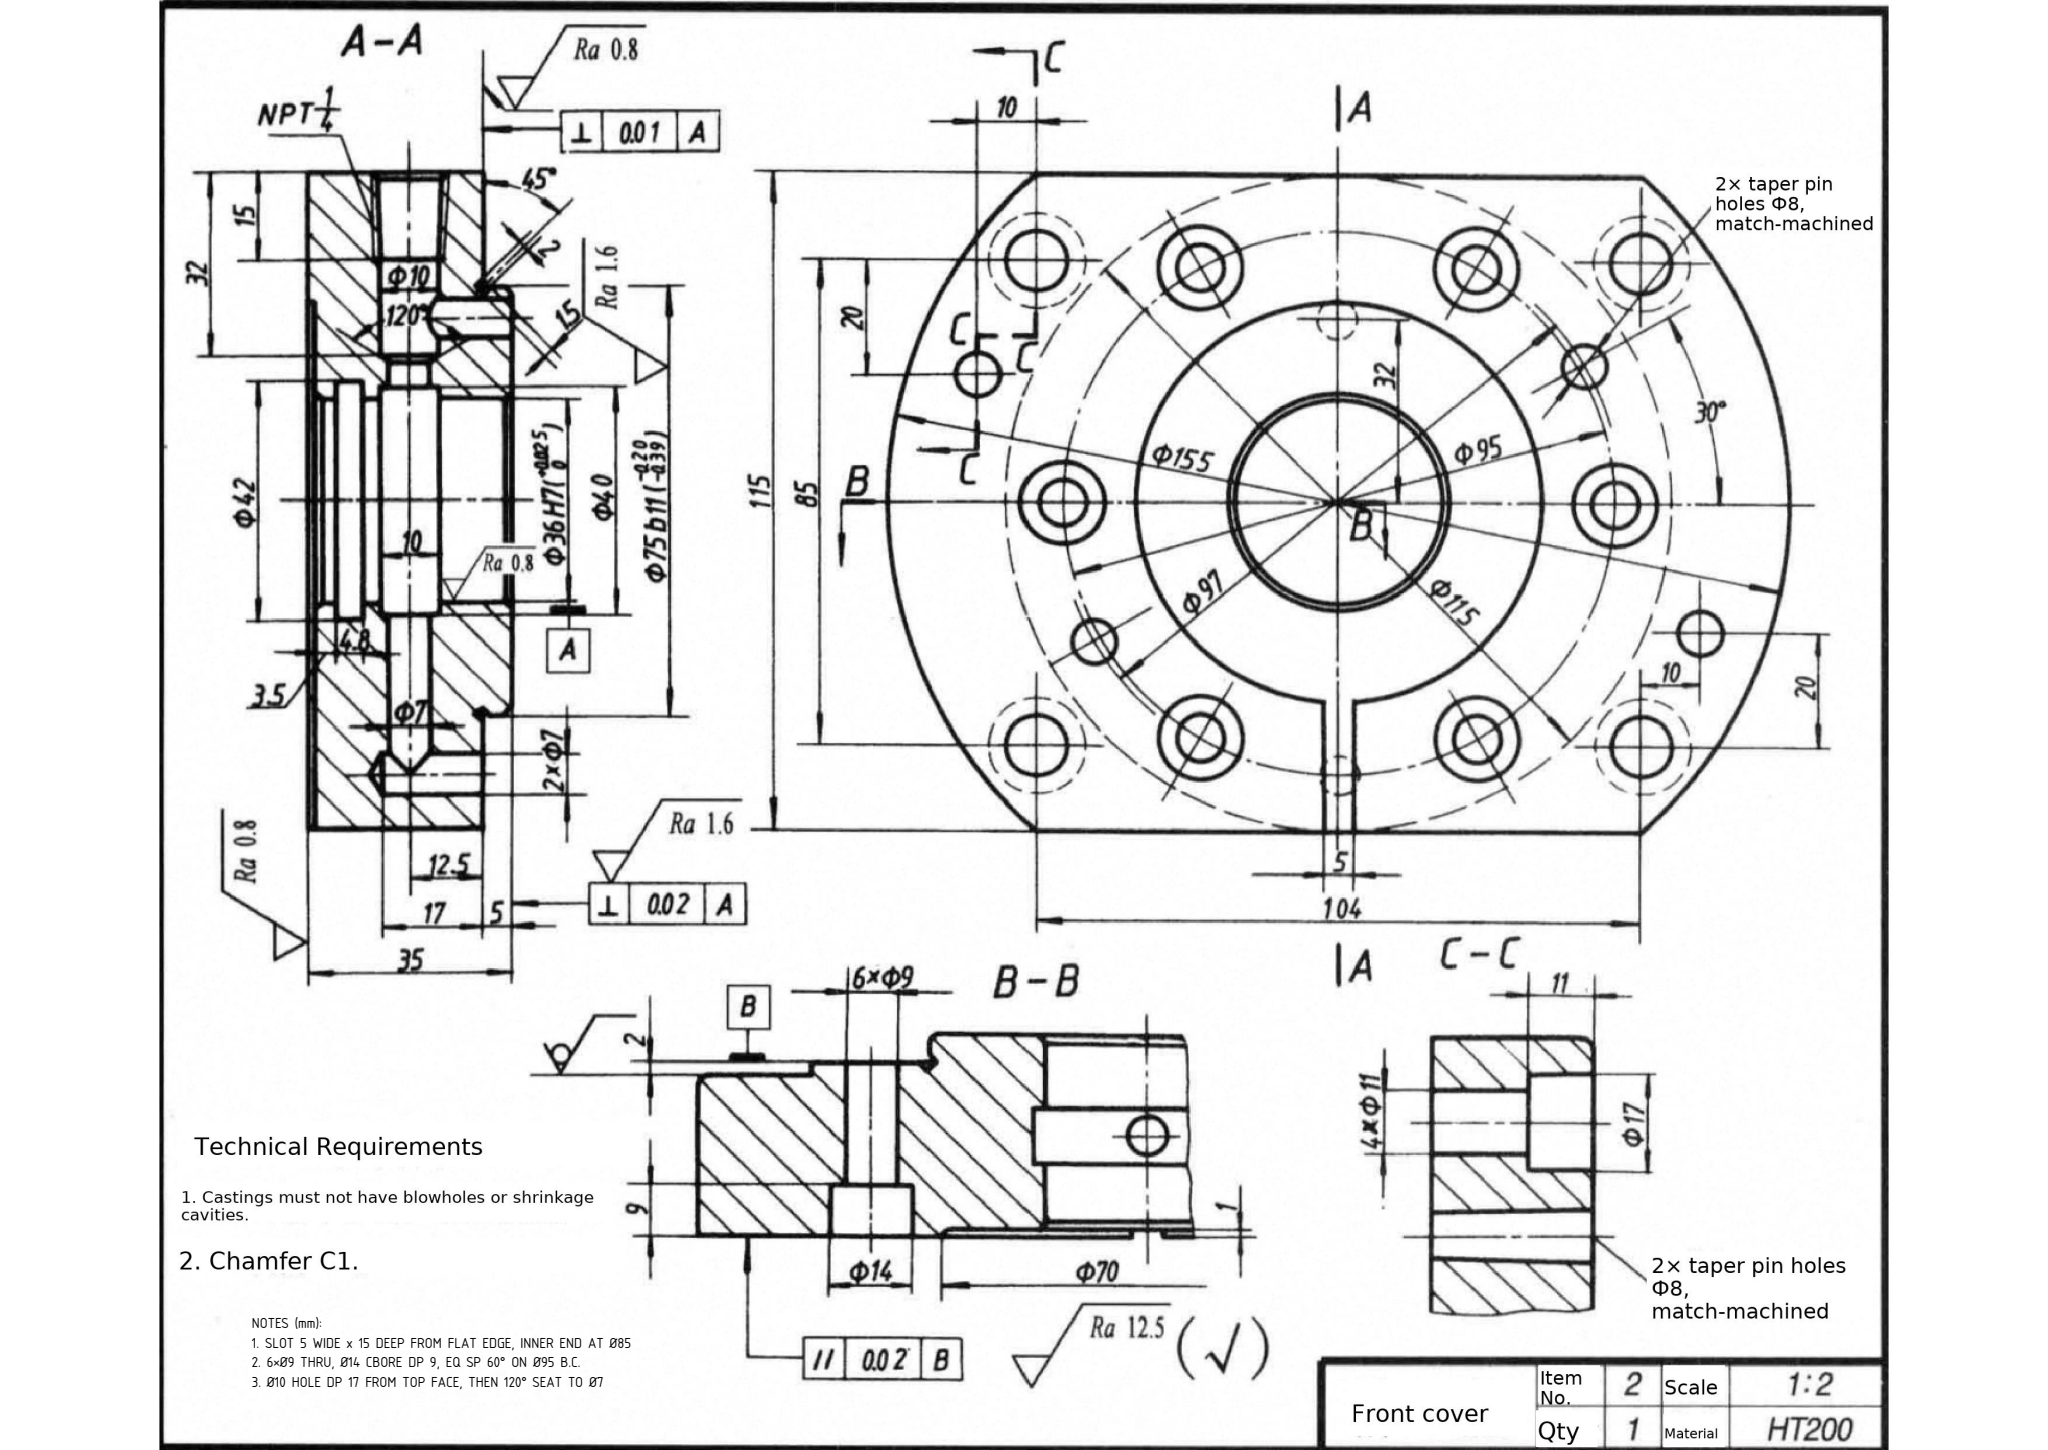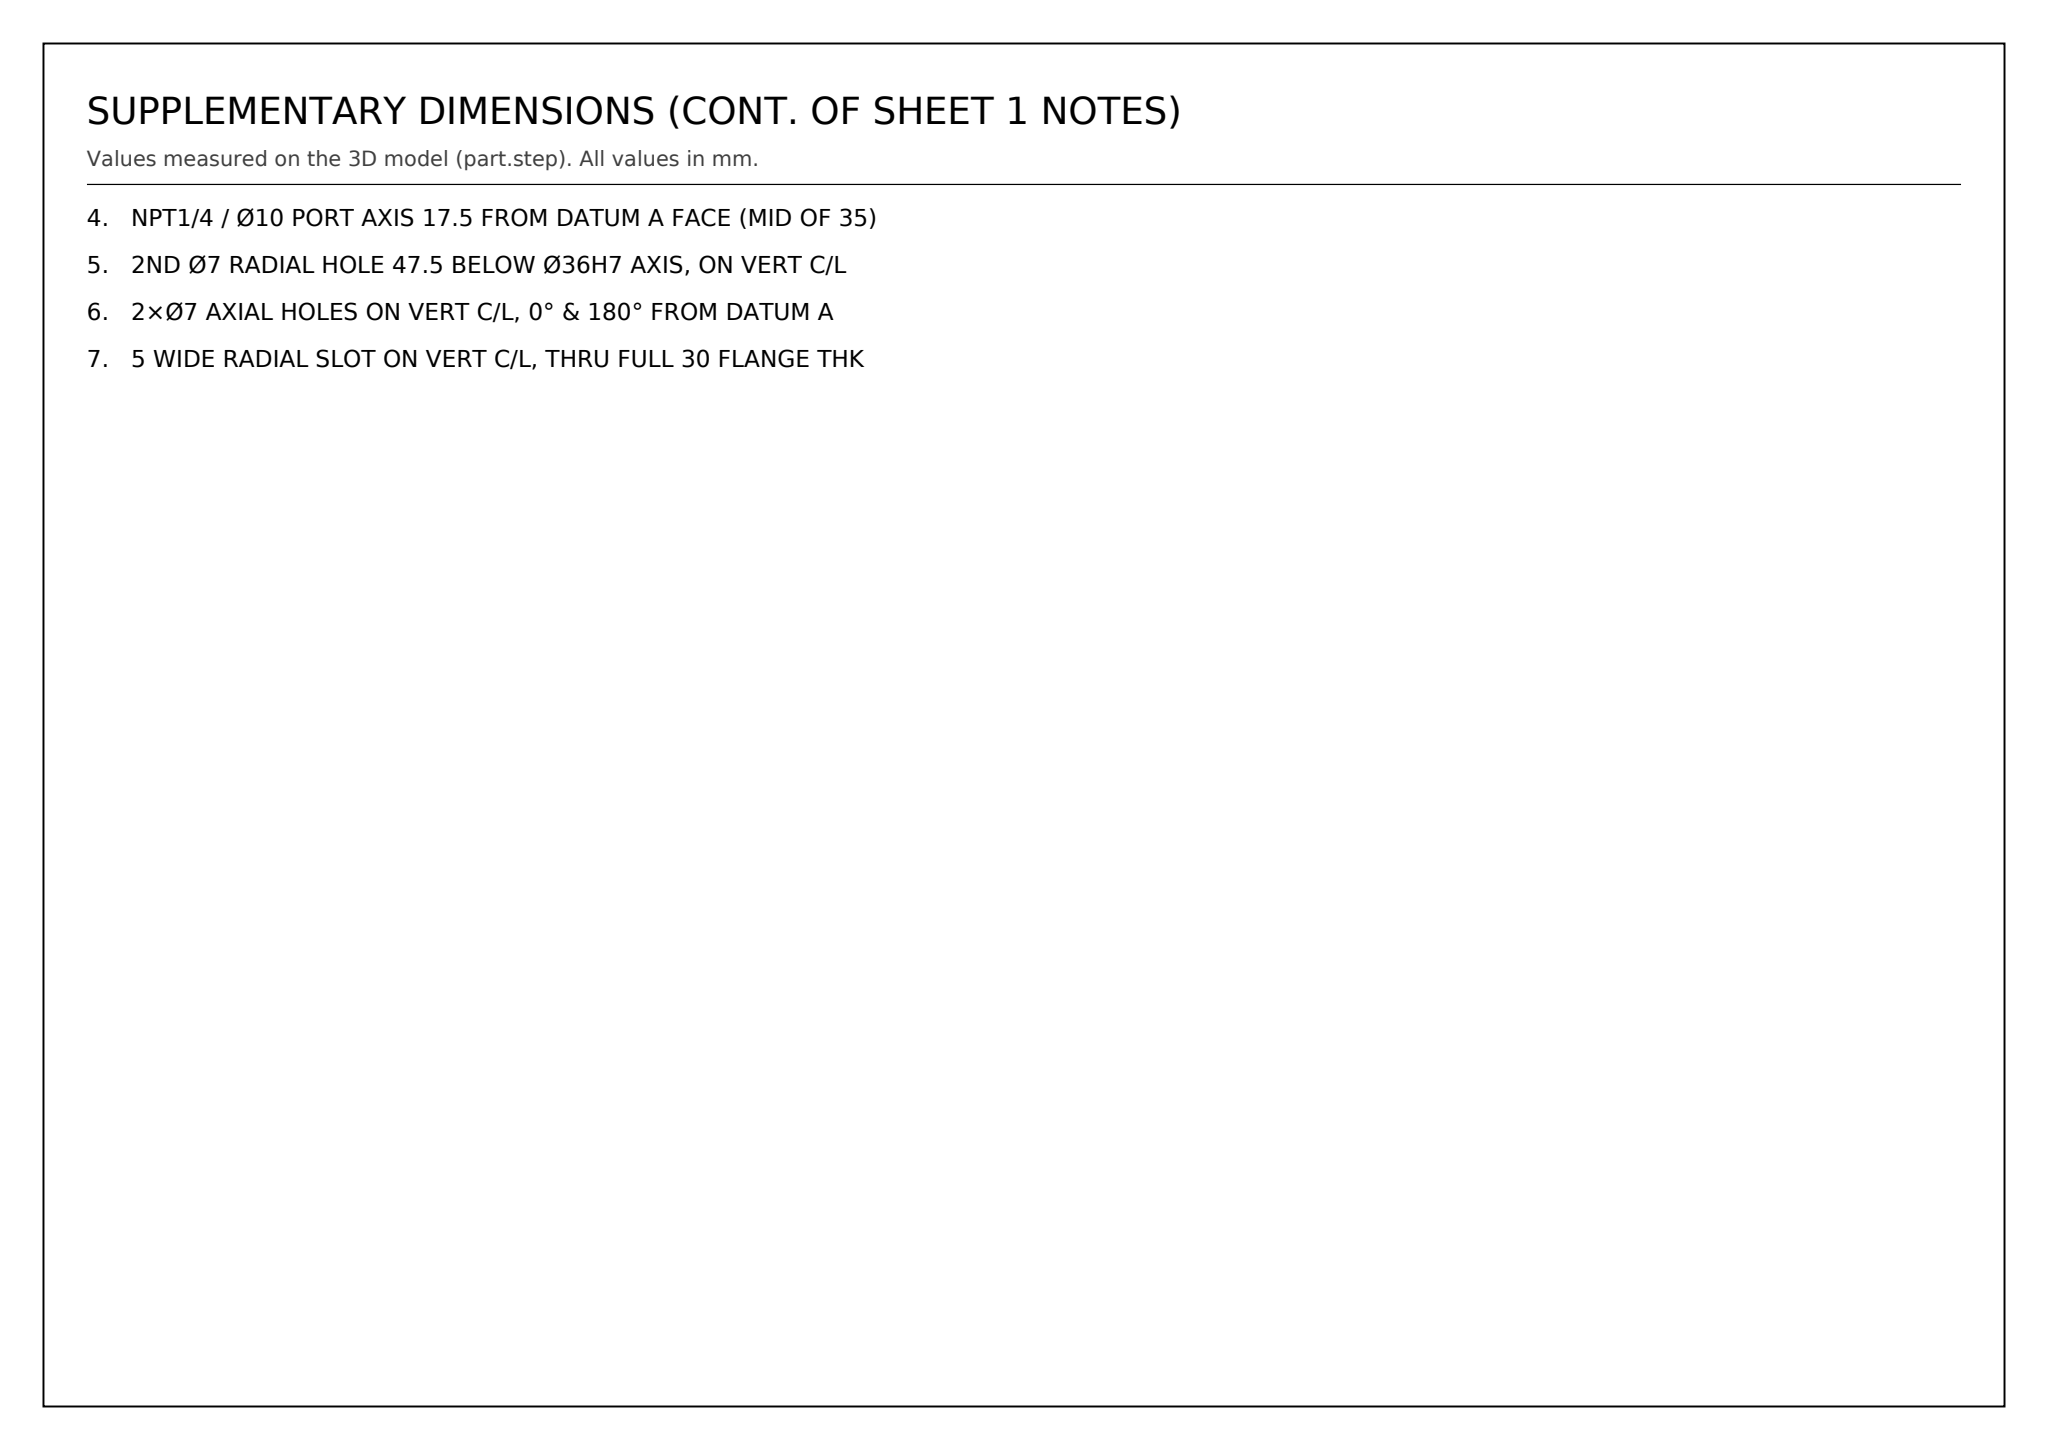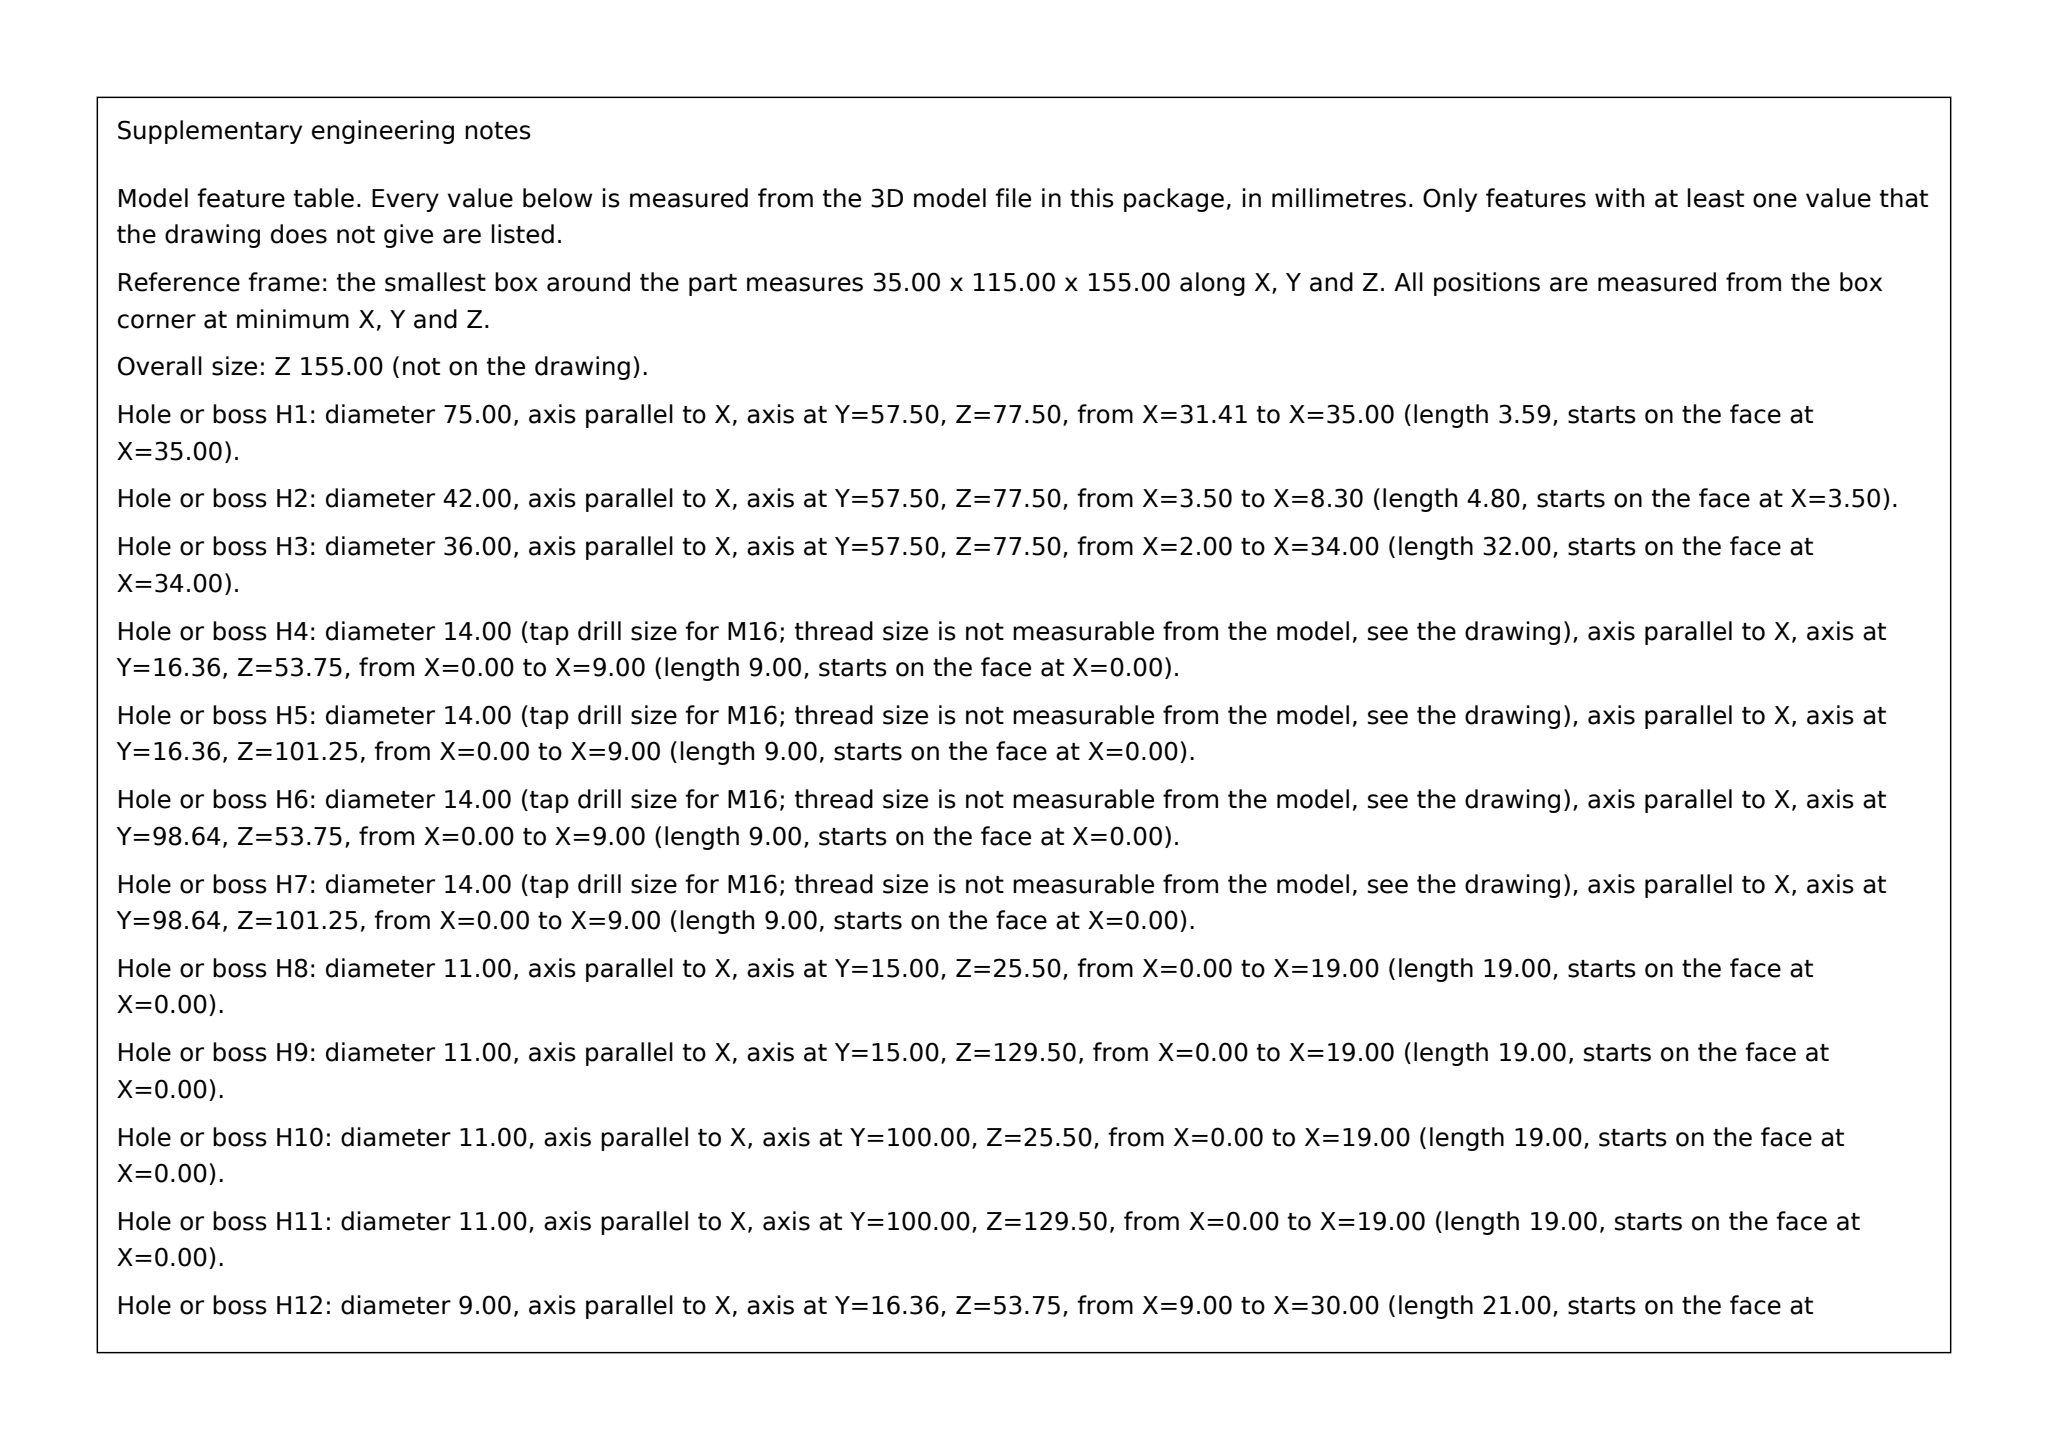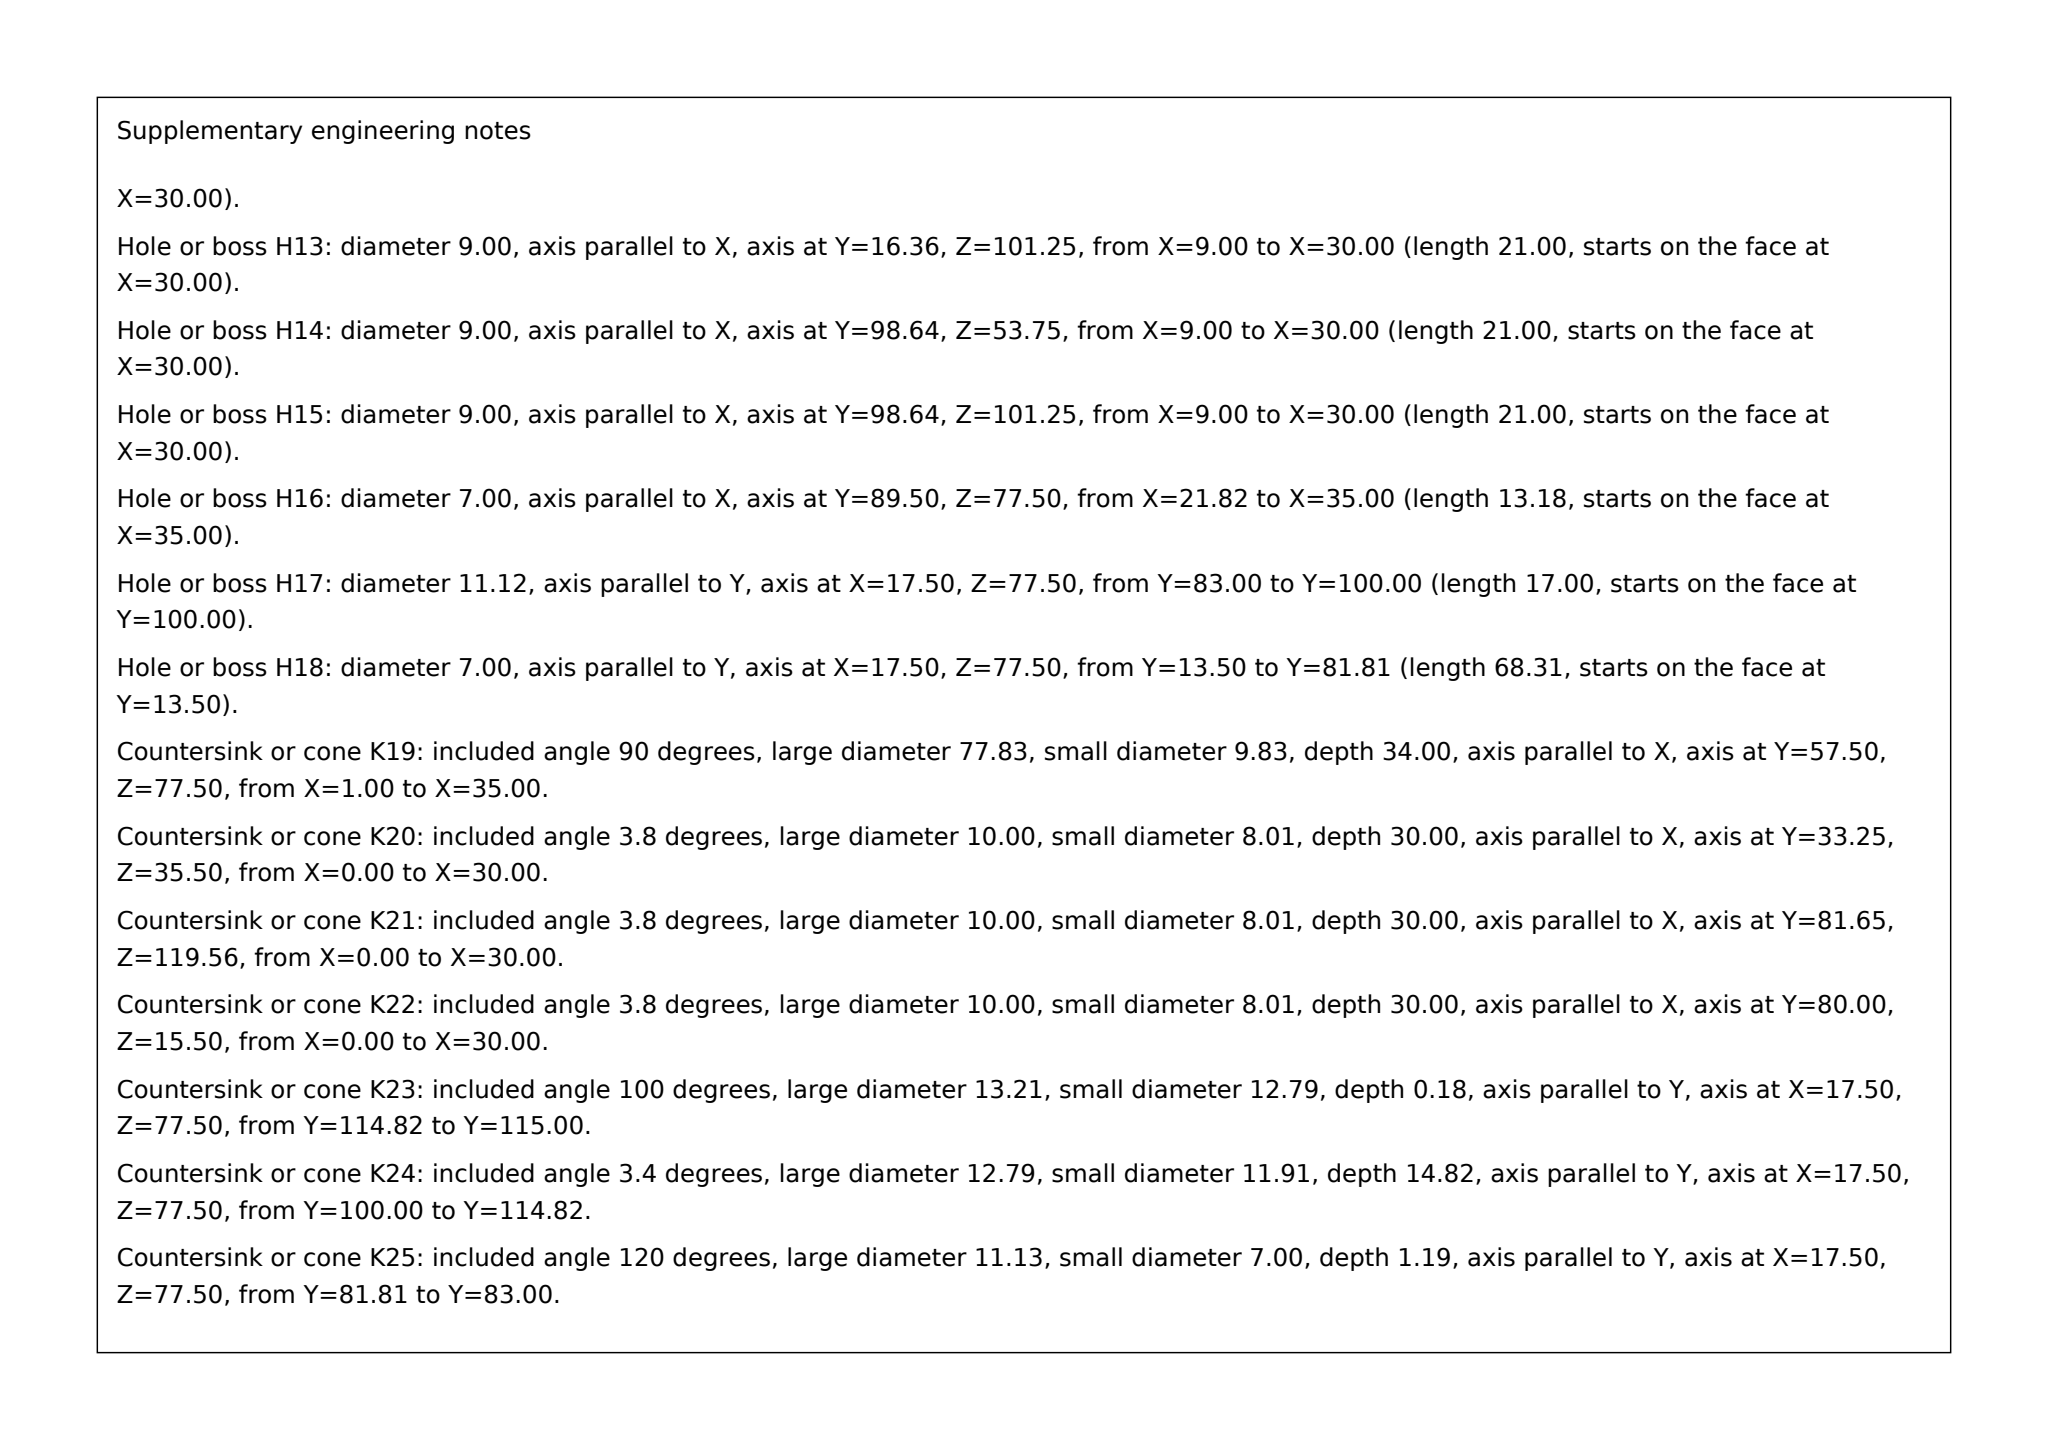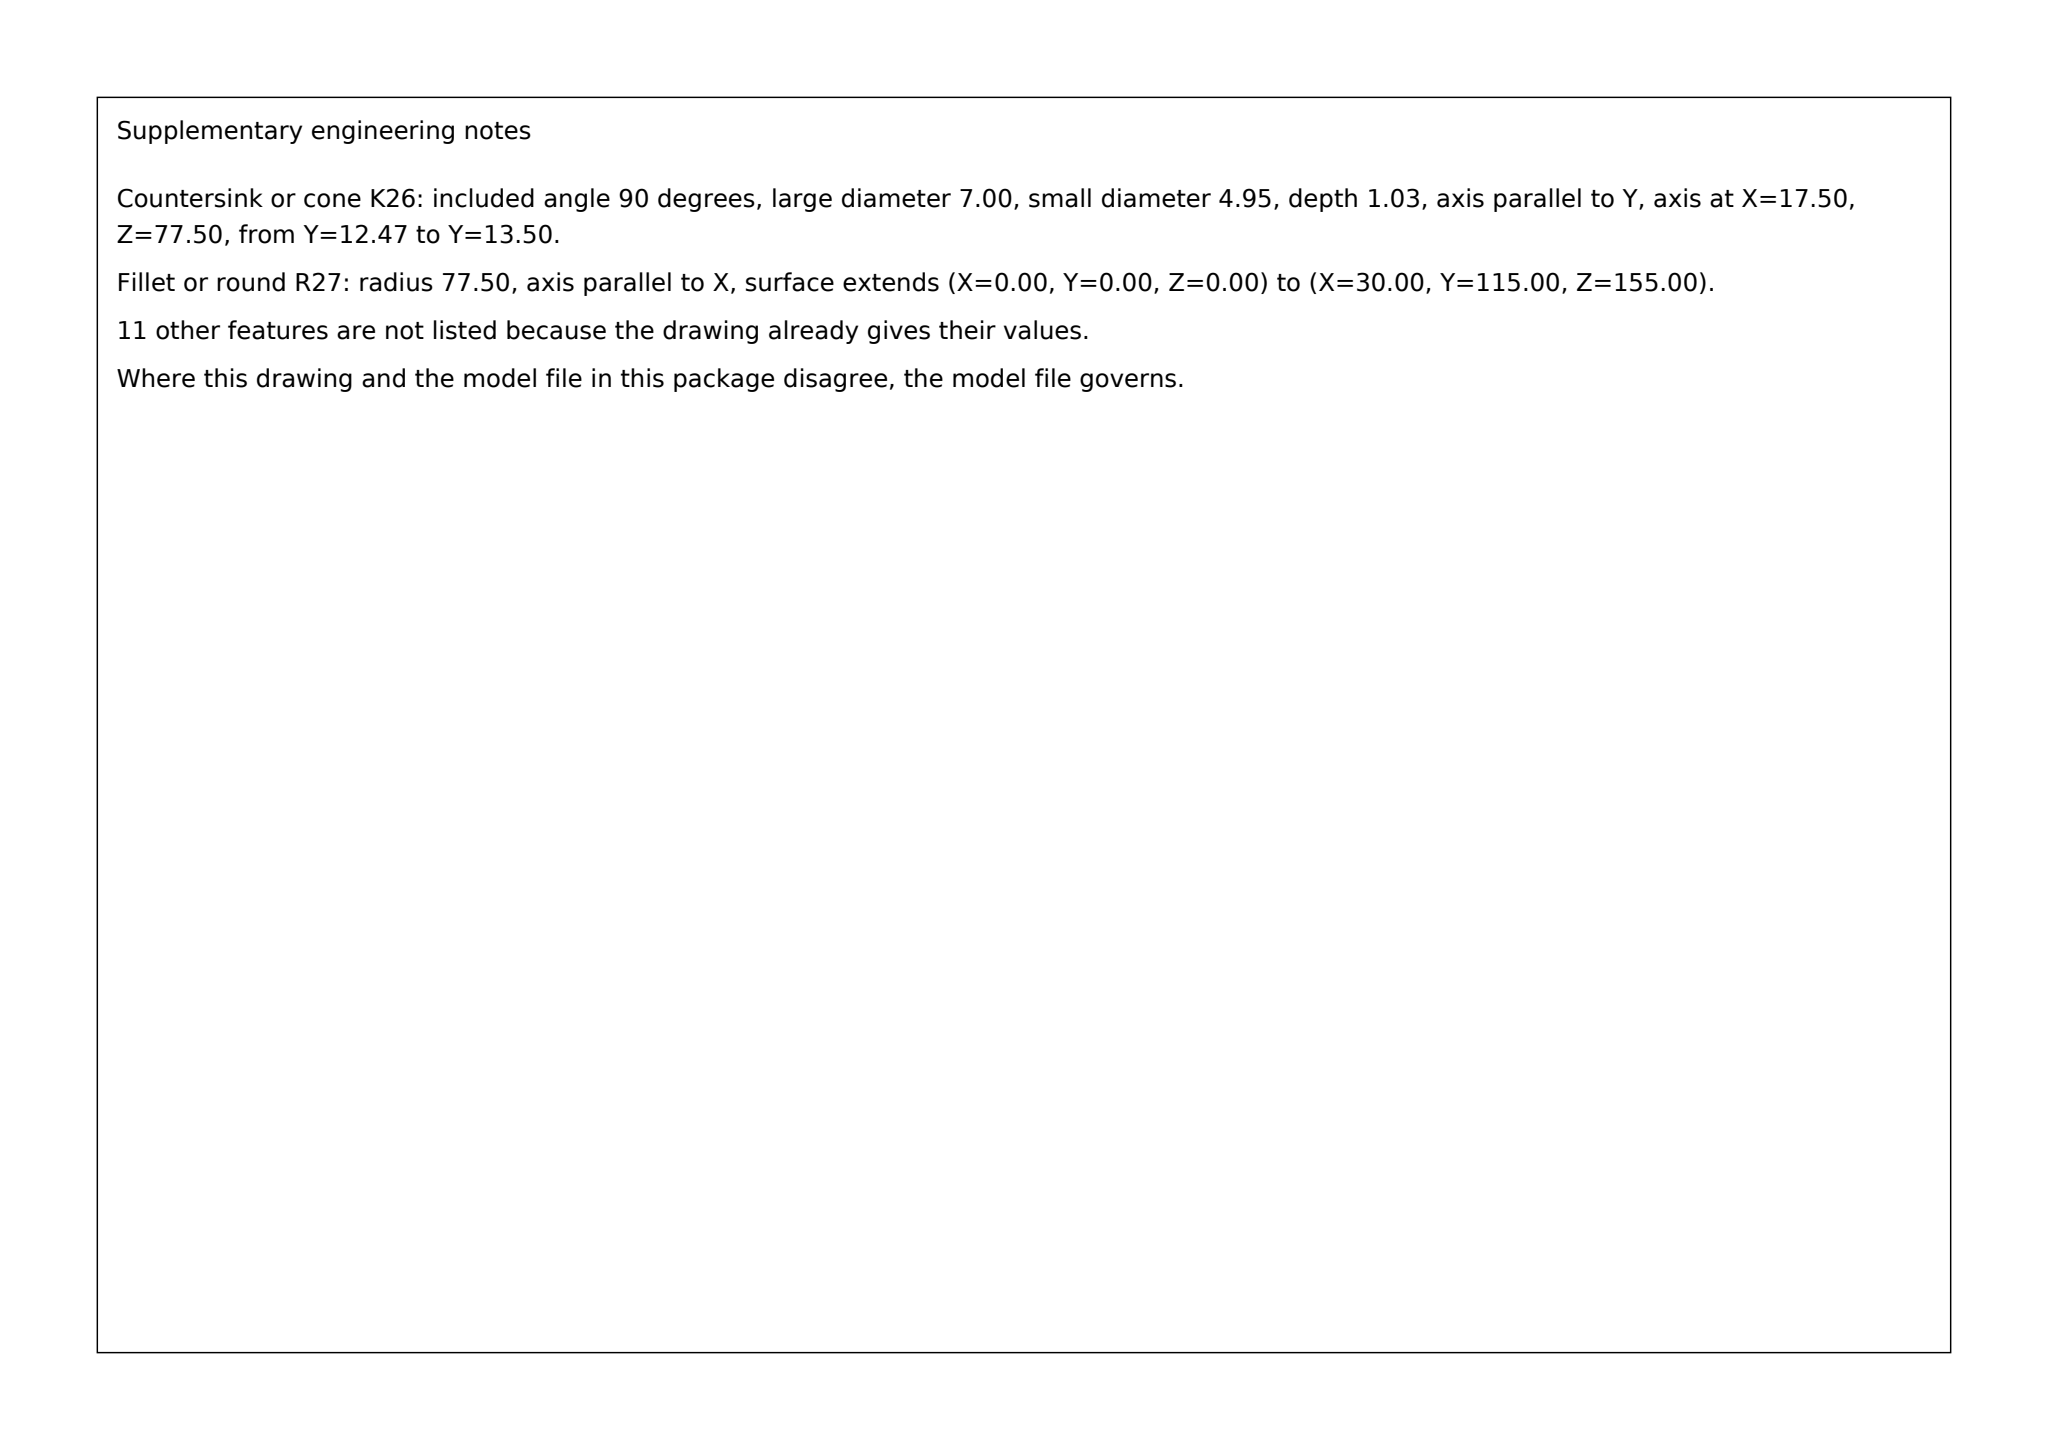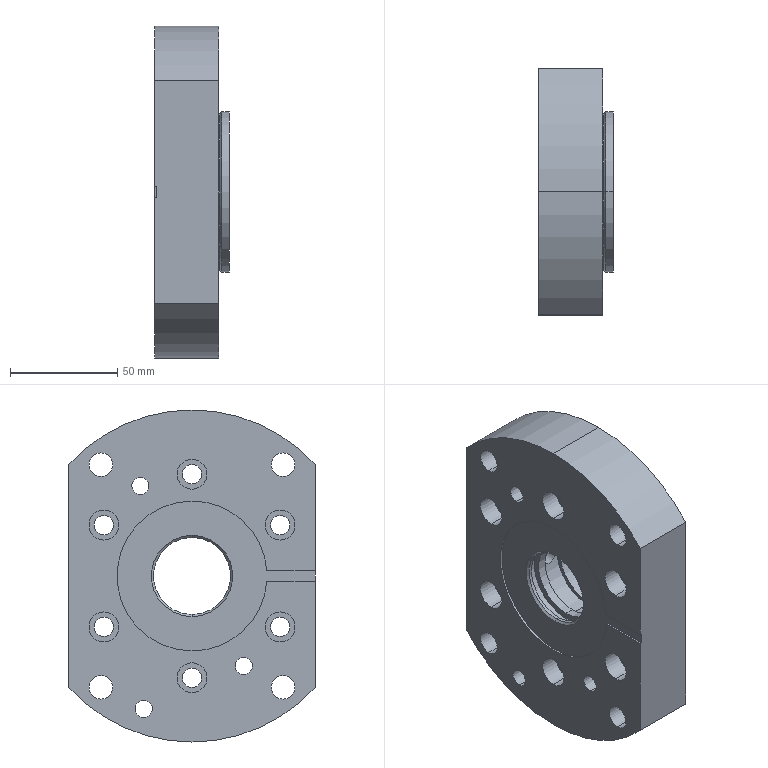Part | SolidWorks | mm | 1 solid | 117 faces | box 35 x 115 x 155 mm | volume 414232 mm3 | cylinder 68 | cone 26 | plane 23 | commonest cylinder face diameters 14 x12 9 x12 17 x8 11 x8 7 x8 36 x6 70 x3 155 x3
Drawing notes:
SLOT 5 WIDE x 15 DEEP FROM FLAT EDGE, INNER END AT Ø85 | from the solid: Slot faces z=75 & z=80 (5 wide, ctr z=77.5); end plane y=100 vs flat y=115 -> 15 deep; r=42.5 from axis y=57.5
6×Ø9 THRU, Ø14 CBORE DP 9, EQ SP 60° ON Ø95 B.C. | from the solid: Ø9 holes at (y,z)=(57.5,30),(16.36,53.75),(16.36,101.25),(57.5,125),(98.64,53.75),(98.64,101.25); all r=47.5 from (57.5,77.5), 60° apart; Ø14 x 9 counterbores
Ø10 HOLE DP 17 FROM TOP FACE, THEN 120° SEAT TO Ø7 | from the solid: Cyl Ø11.125 axis y at (x17.5,z77.5) L=17 from y=115; cone 120° ref dia 11.125 to Ø7 bore
NPT1/4 / Ø10 PORT AXIS 17.5 FROM DATUM A FACE (MID OF 35) | from the solid: Ø11.125 y-axis cyl & 120° cone at x=17.5; part thickness 35 (x 0-35)
2ND Ø7 RADIAL HOLE 47.5 BELOW Ø36H7 AXIS, ON VERT C/L | from the solid: Ø7 x-axis cyls at y=10.0 & y=89.5, z=77.5; bore axis y=57.5 -> 47.5 and 32
2×Ø7 AXIAL HOLES ON VERT C/L, 0° & 180° FROM DATUM A | from the solid: Ø7 x-axis cyls both at z=77.5 = bore C/L plane (155/2)
5 WIDE RADIAL SLOT ON VERT C/L, THRU FULL 30 FLANGE THK | from the solid: planes z=75 & z=80 (5 wide, centred 77.5); Ø155 OD split into 3 arcs of length 30
build123d program:
from build123d import *

# Parameters (mm, degrees)
CUT_EXTRUDE1_DEPTH            = 116.054
F_8_0MM_DOWEL_PIN_HOLE2_D     = 7
F_8_0MM_DOWEL_PIN_HOLE2_DEPTH = 17
F_8_0MM_DOWEL_PIN_HOLE2_TIP   = 2.103
SKETCH10_R                    = 3.5
CUT_EXTRUDE2_DEPTH            = 17.5
HOLE4_D                       = 11
HOLE4_DEPTH                   = 100
HOLE4_CBORE_D                 = 17
HOLE4_CBORE_DEPTH             = 11
CUT_EXTRUDE3_DEPTH            = 1
CHAMFER1_SIZE                 = 1
HOLE5_D                       = 9
HOLE5_DEPTH                   = 100
HOLE5_CBORE_D                 = 14
HOLE5_CBORE_DEPTH             = 9
HOLE6_AT_2_COUNT              = 2
HOLE6_AT_2_PITCH              = 50.848
HOLE6_AT_3_COUNT              = 2
HOLE6_AT_3_PITCH              = 104.074


with BuildPart() as part:
    # Sketch1 → Revolve1 (revolve)
    with BuildSketch(Plane(origin=(0, 0, 0), x_dir=(1, 0, 0), z_dir=(0, 1, 0)), mode=Mode.PRIVATE) as revolve1_sk:
        Polygon((0, 18), (0, 77.5), (30, 77.5), (30, 38.914), (28.942, 37.856), (28.939, 37.854), (30.354, 36.439), (30.356, 36.442), (31.414, 37.5), (35, 37.5), (35, 18), (22.5, 18), (22.5, 20), (12.5, 20), (12.5, 18), (8.3, 18), (8.3, 21), (3.5, 21), (3.5, 18), align=None)
    revolve(revolve1_sk.sketch.rotate(Axis((-76.834, 0, 0), (1, 0, 0)), 180), axis=Axis((-76.834, 0, 0), (1, 0, 0)))

    # Sketch2 → Cut-Extrude1 (cut, through all)
    with BuildSketch(Plane.ZY):
        with BuildLine():
            Line((-51.962, 57.5), (51.962, 57.5))
            ThreePointArc((51.962, 57.5), (0, 77.5), (-51.962, 57.5))
        make_face()
        with BuildLine():
            Line((-51.962, -57.5), (51.962, -57.5))
            ThreePointArc((51.962, -57.5), (0, -77.5), (-51.962, -57.5))
        make_face()
    extrude(amount=-CUT_EXTRUDE1_DEPTH, mode=Mode.SUBTRACT)

    # Sketch7 → Cut-Revolve1 (revolve, cut)
    with BuildSketch(Plane.XY):
        Polygon((17.5, 57.5), (17.5, -47.5), (14, -44), (14, 57.5), align=None)
    revolve(axis=Axis((17.5, 57.5, 0), (0, -1, 0)), mode=Mode.SUBTRACT)

    # 8.0mm Dowel Pin Hole2
    with Locations(Plane(origin=(30, 0, 0), x_dir=(0, 0, -1), z_dir=(1, 0, 0))):
        with Locations((0, -47.5)):
            Hole(F_8_0MM_DOWEL_PIN_HOLE2_D / 2, depth=F_8_0MM_DOWEL_PIN_HOLE2_DEPTH)
            with Locations((0, 0, -(F_8_0MM_DOWEL_PIN_HOLE2_DEPTH + F_8_0MM_DOWEL_PIN_HOLE2_TIP / 2))):  # 118° drill point
                Cone(0, F_8_0MM_DOWEL_PIN_HOLE2_D / 2, F_8_0MM_DOWEL_PIN_HOLE2_TIP, mode=Mode.SUBTRACT)

    # Sketch10 → Cut-Extrude2 (cut)
    with BuildSketch(Plane(origin=(35, 0, 0), x_dir=(0, 0, -1), z_dir=(1, 0, 0))):
        with Locations((0, 32)):
            Circle(SKETCH10_R)
    extrude(amount=-CUT_EXTRUDE2_DEPTH, mode=Mode.SUBTRACT)

    # Hole4
    with Locations(Plane(origin=(30, 0, 0), x_dir=(0, 0, -1), z_dir=(1, 0, 0))):
        with Locations((52, 42.5), (-52, 42.5), (52, -42.5), (-52, -42.5)):
            CounterBoreHole(HOLE4_D / 2, HOLE4_CBORE_D / 2, HOLE4_CBORE_DEPTH, depth=HOLE4_DEPTH)

    # Sketch15 → Cut-Extrude3 (cut)
    with BuildSketch(Plane.ZY):
        with BuildLine():
            Line((-2.5, -34.911), (-2.5, -57.5))
            Line((-2.5, -57.5), (2.5, -57.5))
            Line((2.5, -57.5), (2.5, -34.911))
            ThreePointArc((2.5, -34.911), (0, 35), (-2.5, -34.911))
        make_face()
    extrude(amount=-CUT_EXTRUDE3_DEPTH, mode=Mode.SUBTRACT)

    # Chamfer1
    chamfer1_edges = [part.edges().sort_by_distance(p)[0] for p in [
        (1, 0, -18),
        (35, 0, -18),
    ]]
    chamfer(chamfer1_edges, length=CHAMFER1_SIZE)

    # Sketch17 → 1_4 NPT Tapped Hole1 (revolve, cut)
    with BuildSketch(Plane(origin=(17.5, 57.5, 0), x_dir=(0, 0, 1), z_dir=(1, 0, 0))):
        Polygon((0, 0), (0, 35.212), (5.563, 32), (5.563, 15), (5.949, 15), (6.393, 0.1772), (6.604, 0), align=None)
    revolve(axis=Axis((17.5, 63.85, 0), (0, -1, 0)), mode=Mode.SUBTRACT)

    # Hole5
    with Locations(Plane(origin=(0, 41.136, -23.75), x_dir=(0, 0, -1), z_dir=(-1, 0, 0))):
        with Locations((0, 0), (-47.5, 0), (-71.25, 41.136), (23.75, 41.136), (0, 82.272), (-47.5, 82.272)):
            CounterBoreHole(HOLE5_D / 2, HOLE5_CBORE_D / 2, HOLE5_CBORE_DEPTH, depth=HOLE5_DEPTH)

    # Sketch20 → Hole6 (revolve, cut)
    with BuildSketch(Plane(origin=(0, 22.5, -62), x_dir=(0, 0, 1), z_dir=(0, 1, 0))):
        Polygon((0, 0), (0, 30), (5, 30), (4, 0), align=None)
    hole6 = revolve(axis=Axis((110, 22.5, -62), (-1, 0, 0)), mode=Mode.SUBTRACT)

    # Hole6 at 2: Hole6 ×2
    with Locations(*[Vector(0, -0.9194, 0.3933) * (i * HOLE6_AT_2_PITCH) for i in range(1, HOLE6_AT_2_COUNT)]):
        add(hole6, mode=Mode.SUBTRACT)

    # Hole6 at 3: Hole6 ×2
    with Locations(*[Vector(0, 0.01584, 0.9999) * (i * HOLE6_AT_3_PITCH) for i in range(1, HOLE6_AT_3_COUNT)]):
        add(hole6, mode=Mode.SUBTRACT)


solid = part.part